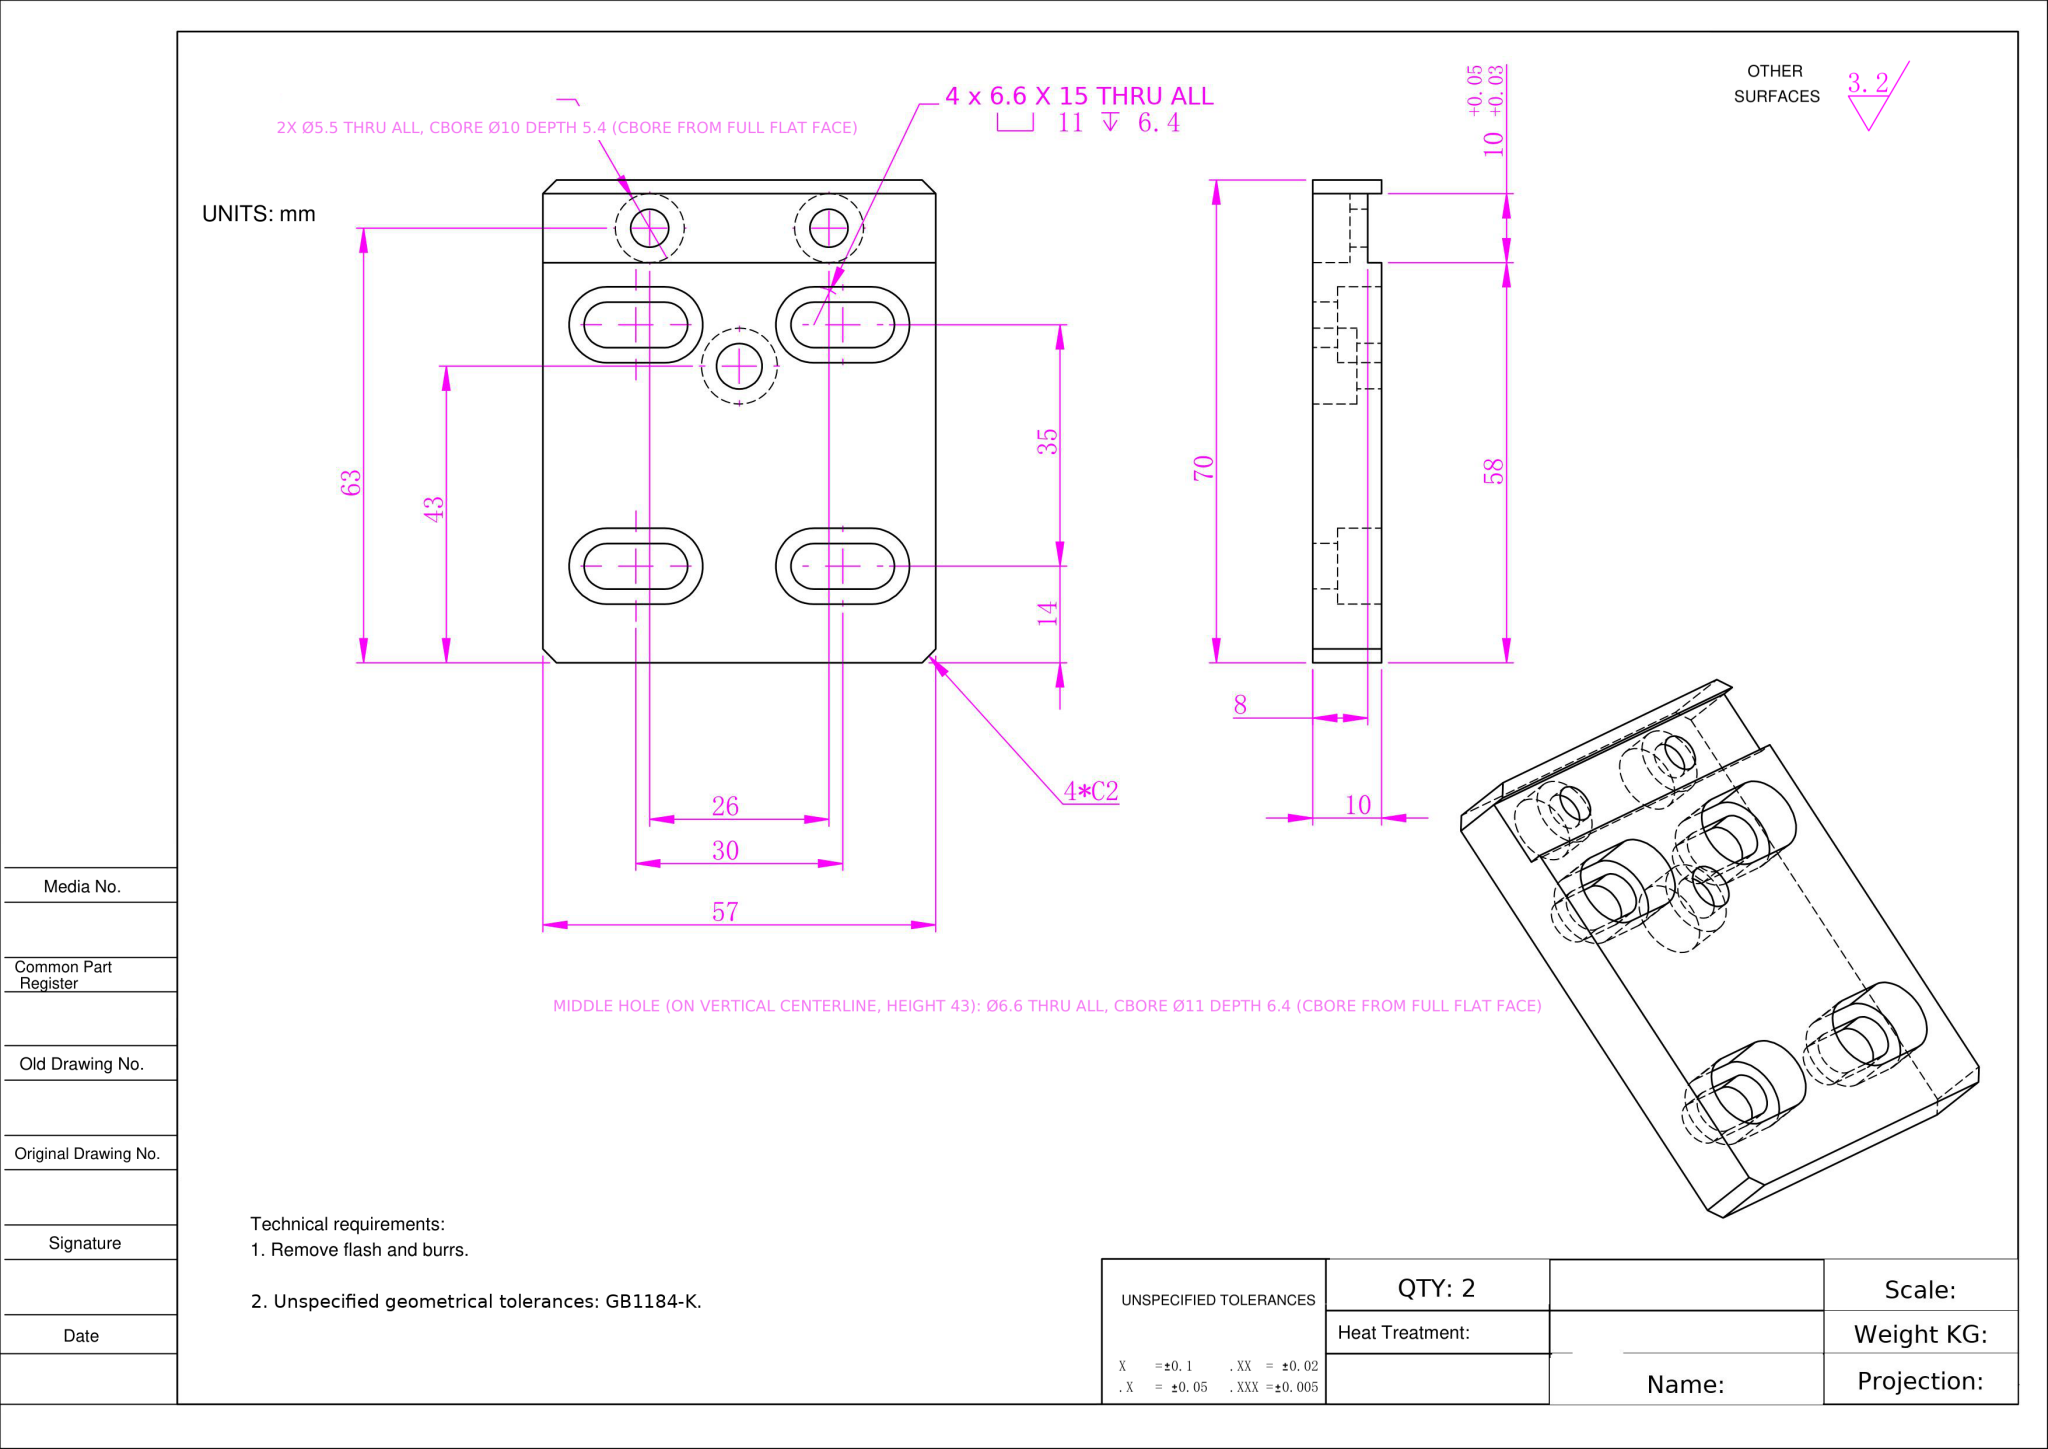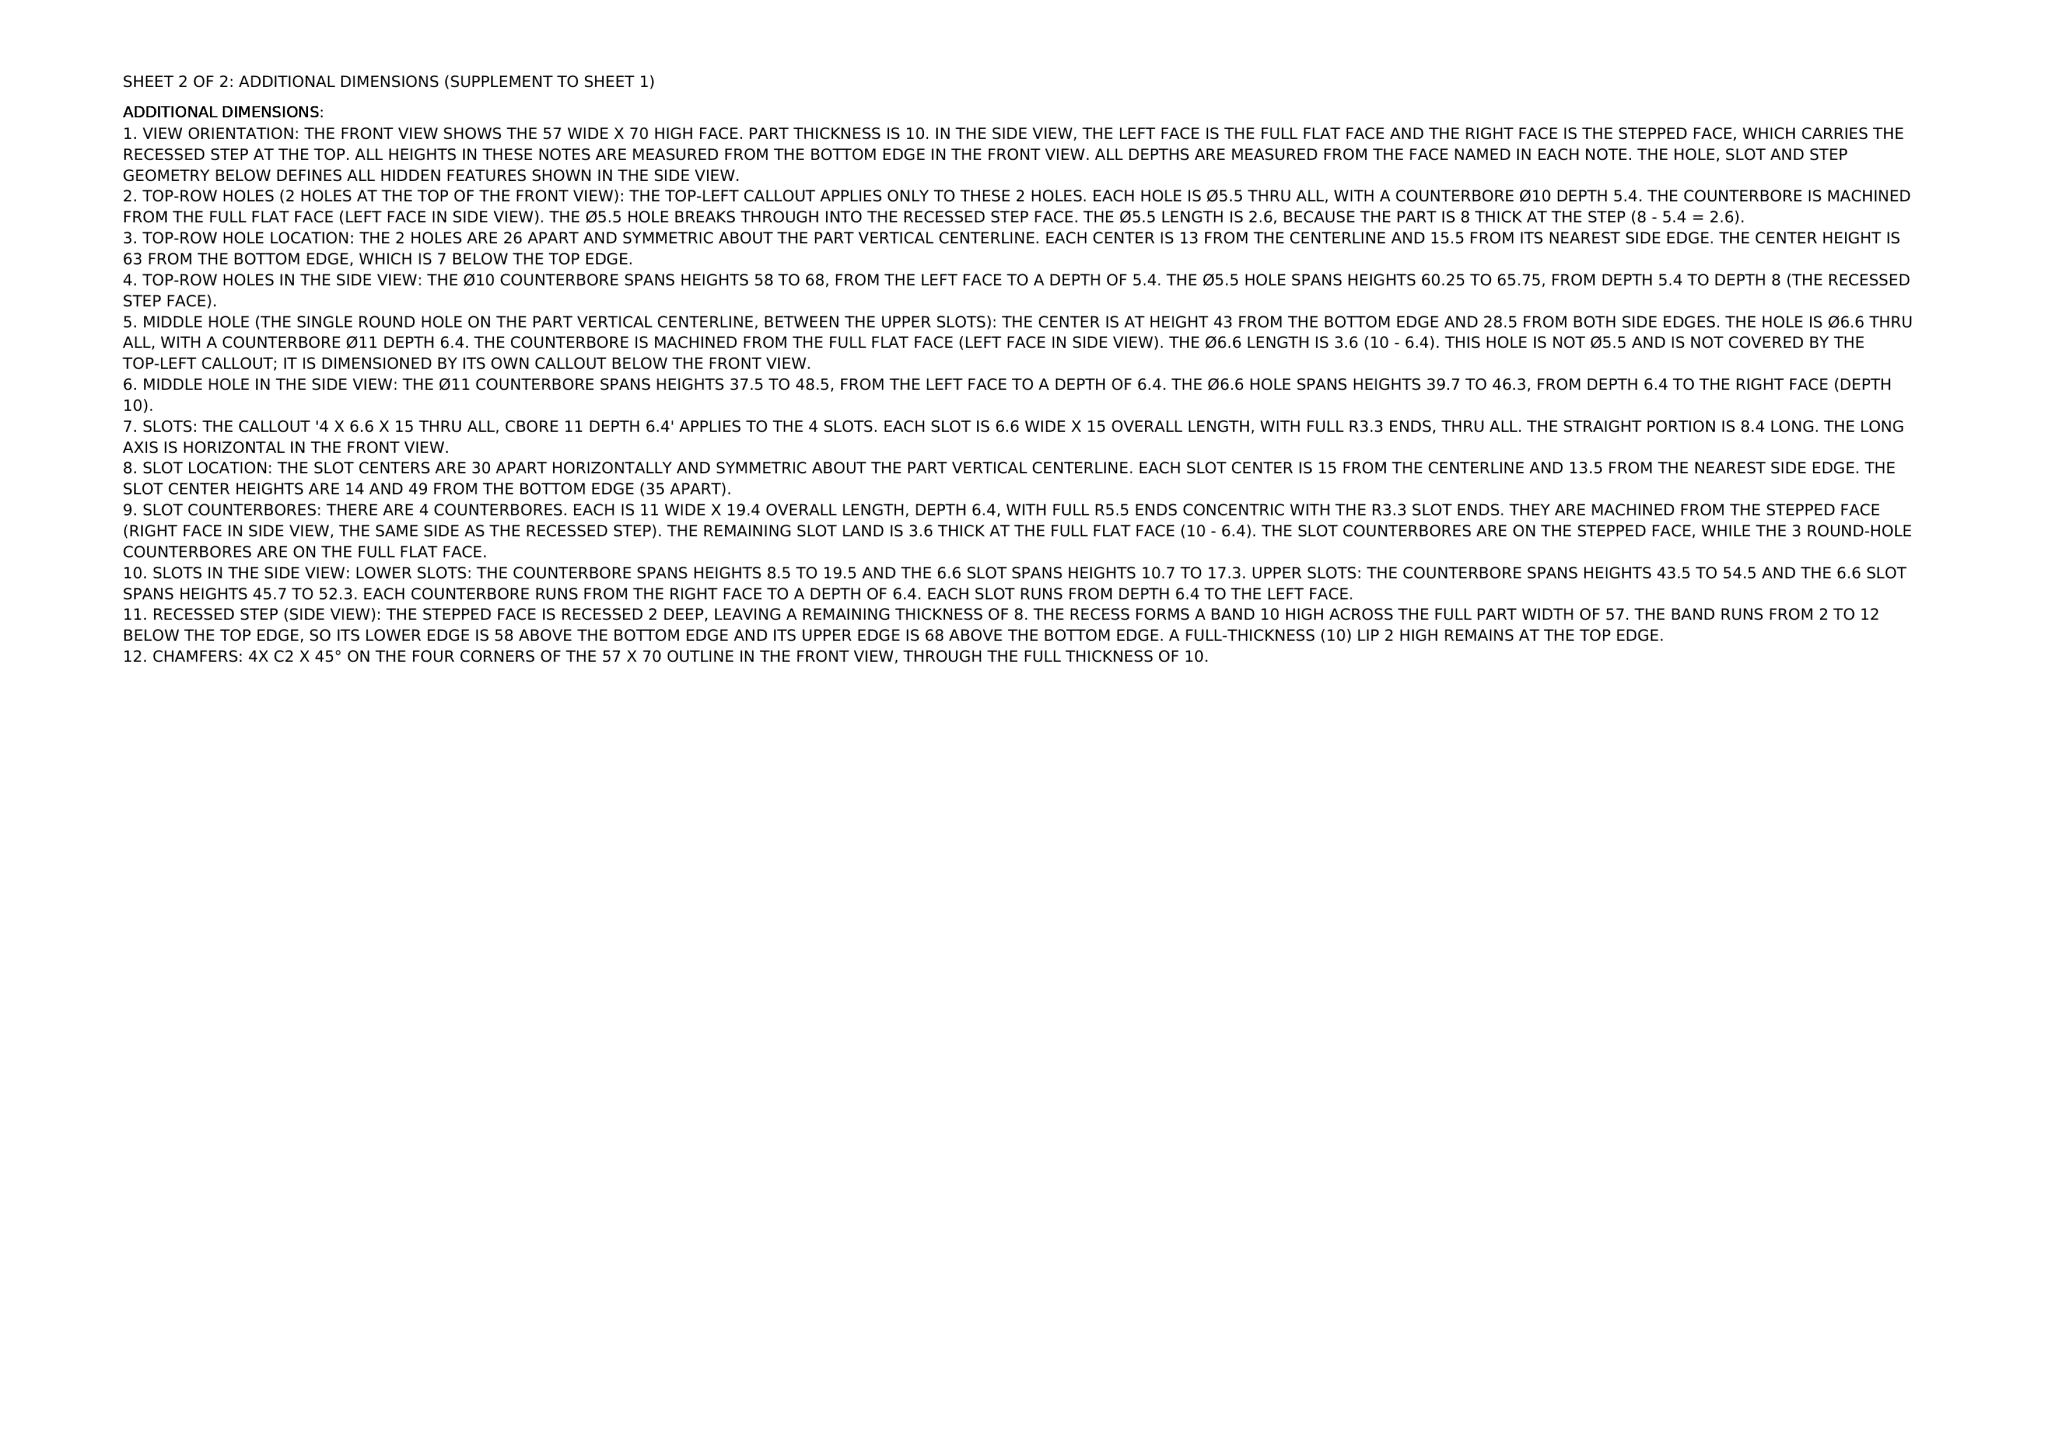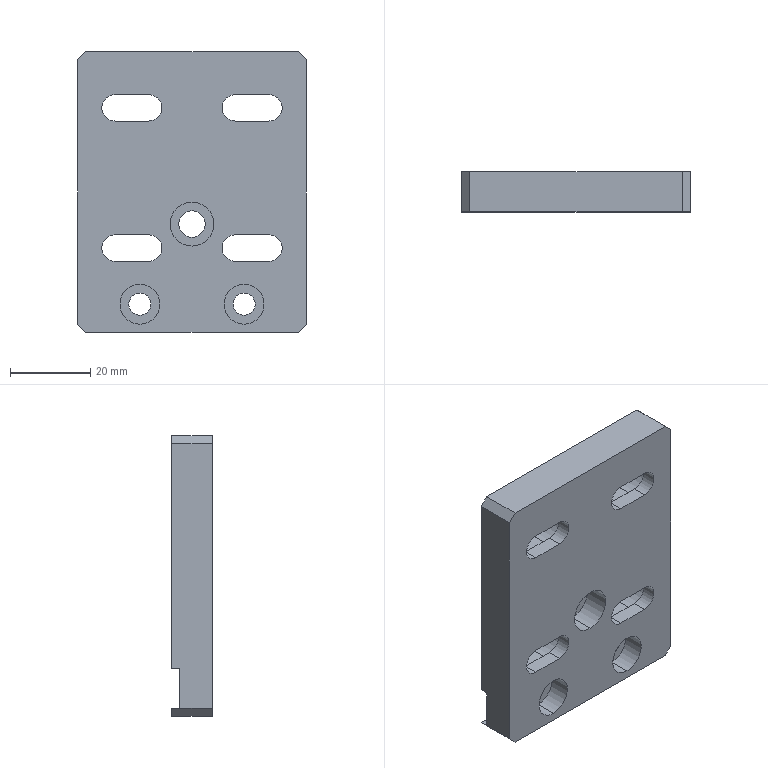Part | NX | mm | 1 solid | 65 faces | box 57 x 10 x 70 mm | volume 30888 mm3 | plane 37 | cylinder 28 | commonest cylinder face diameters 11 x10 6.6 x10 10 x4 5.5 x4